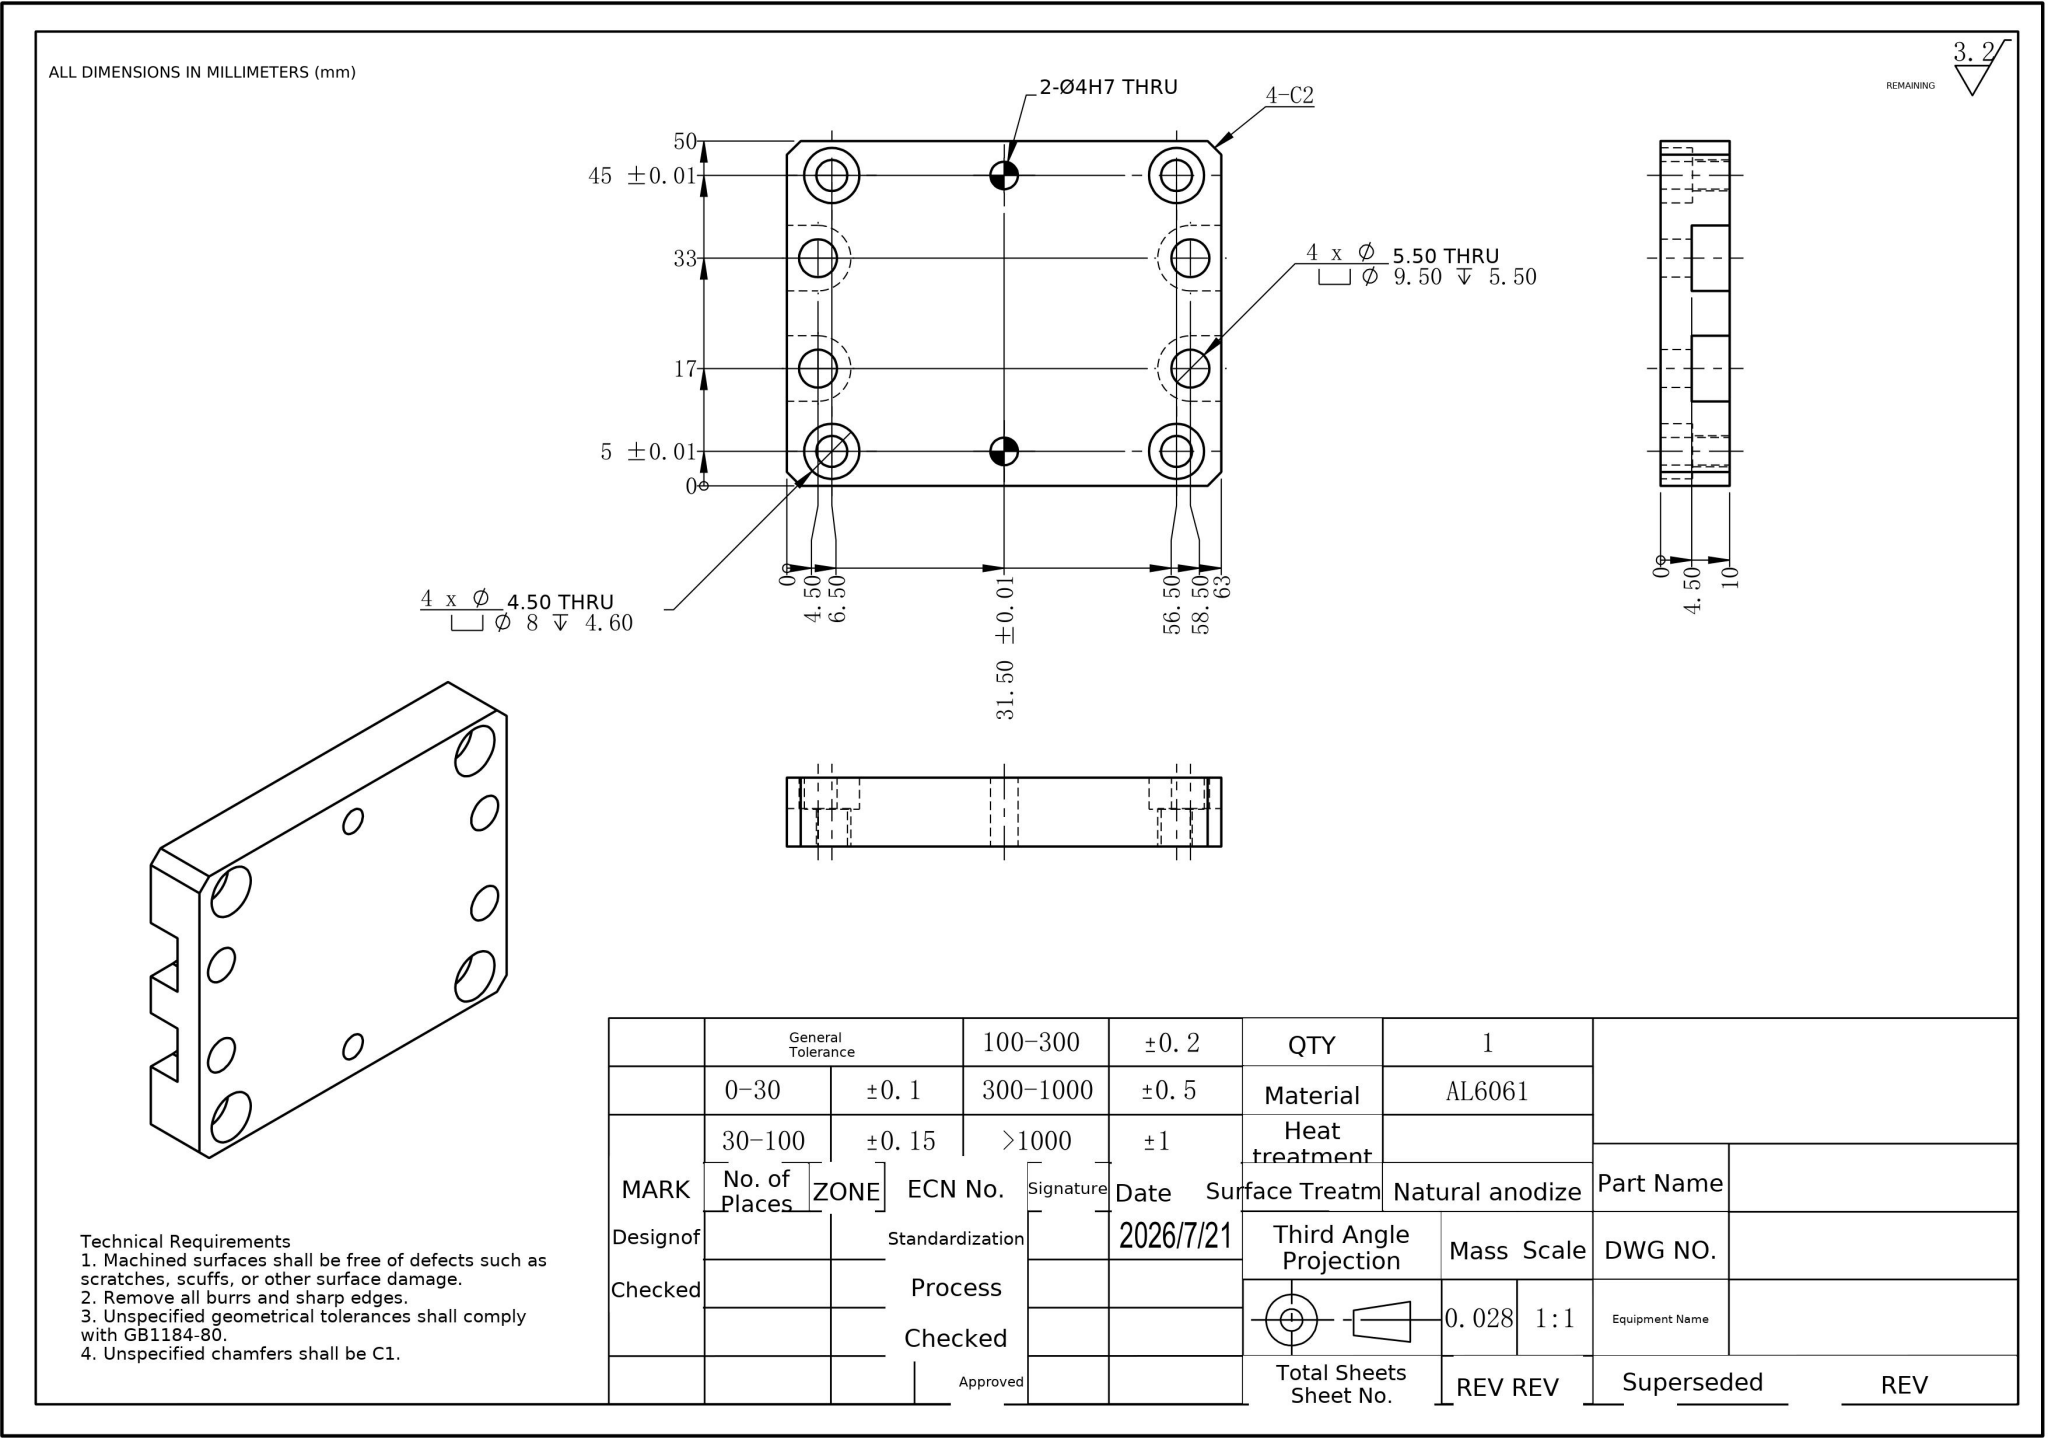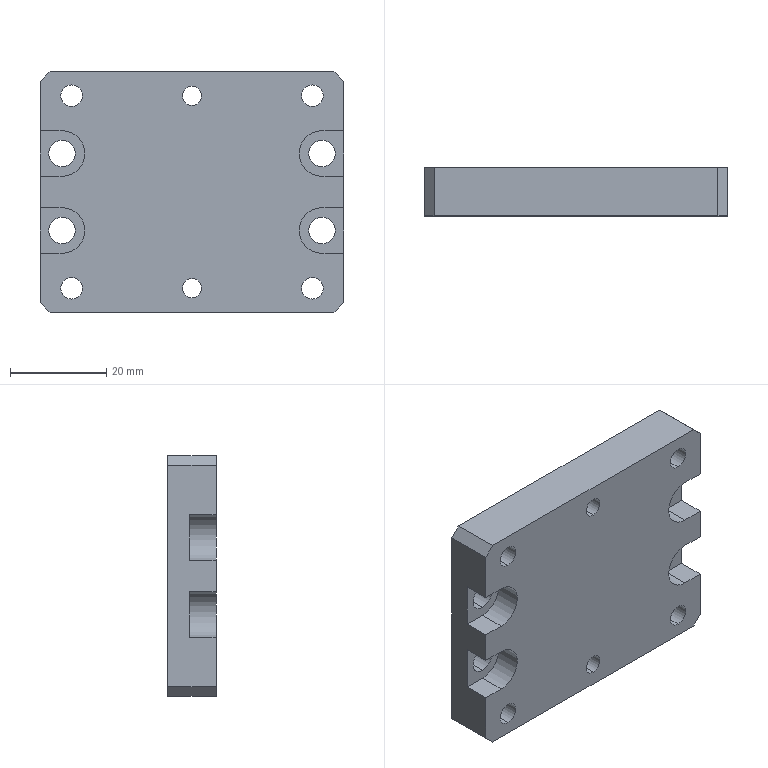Part | NX | mm | 1 solid | 58 faces | box 63 x 10 x 50 mm | volume 27752 mm3 | cylinder 32 | plane 26 | commonest cylinder face diameters 5.5 x8 8 x8 4.5 x8 4 x4 9.5 x4